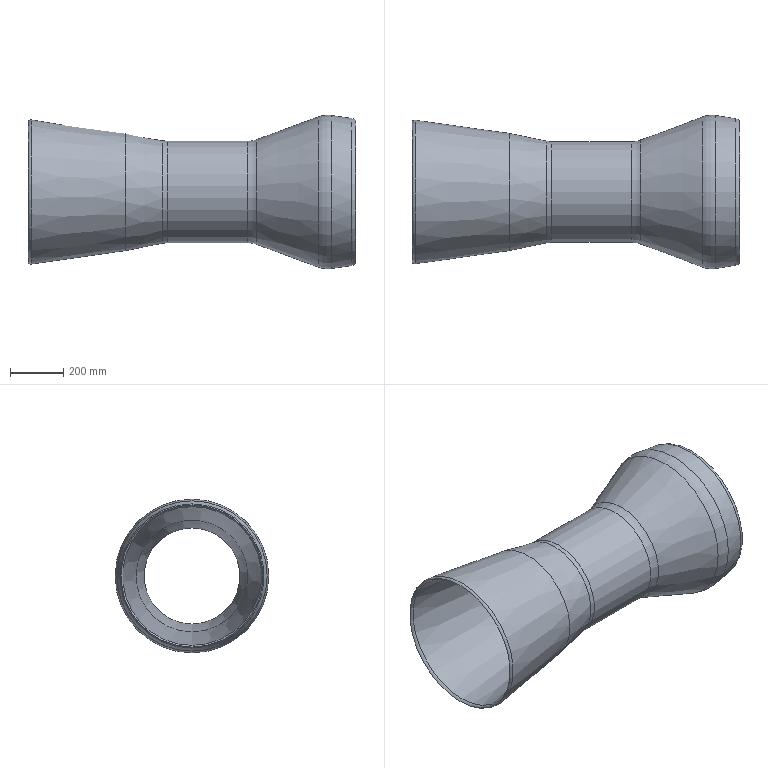Component | NX | HOUSING | 1 solid | 17 faces | volume 17352414 mm3 | cone 8 | torus 7 | cylinder 2 | commonest cylinder face diameters 360 x1 380 x1